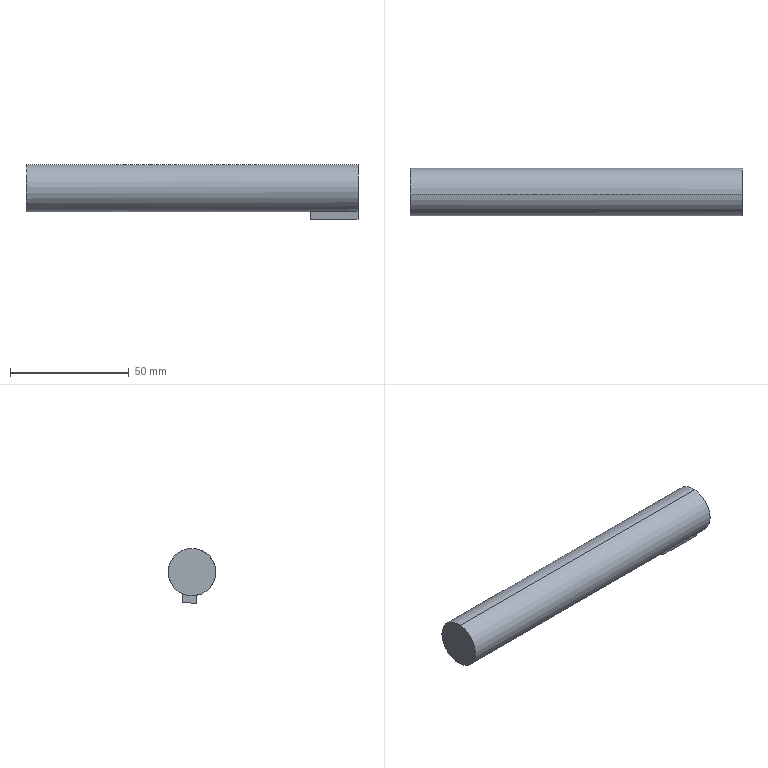Component | SolidWorks | ArmServoMotorAssembly-1_ArmServoMotorAxis-1 | 1 solid | 8 faces | box 140 x 20 x 23.22 mm | volume 44361 mm3 | plane 6 | cylinder 2 | commonest cylinder face diameters 20 x2
build123d program:
from build123d import *

# Parameters (mm, degrees)
SKETCH1_R           = 10
BOSS_EXTRUDE1_DEPTH = 140
SKETCH3_W           = 20
SKETCH3_H           = 6
BOSS_EXTRUDE2_DEPTH = 5


with BuildPart() as part:
    # Sketch1 → Boss-Extrude1 (new body)
    with BuildSketch(Plane.XY):
        Circle(SKETCH1_R)
    extrude(amount=BOSS_EXTRUDE1_DEPTH)

    # Sketch3 → Boss-Extrude2 (add)
    with BuildSketch(Plane(origin=(8, 0, 0), x_dir=(0, 0, -1), z_dir=(1, 0, 0))):
        with Locations((-10, 0)):
            Rectangle(SKETCH3_W, SKETCH3_H)
    extrude(amount=BOSS_EXTRUDE2_DEPTH)


solid = part.part

# Placed as in the assembly
solid = solid.moved(Location((105.641, 70.663, 0), (-174.806, -90, 0)))